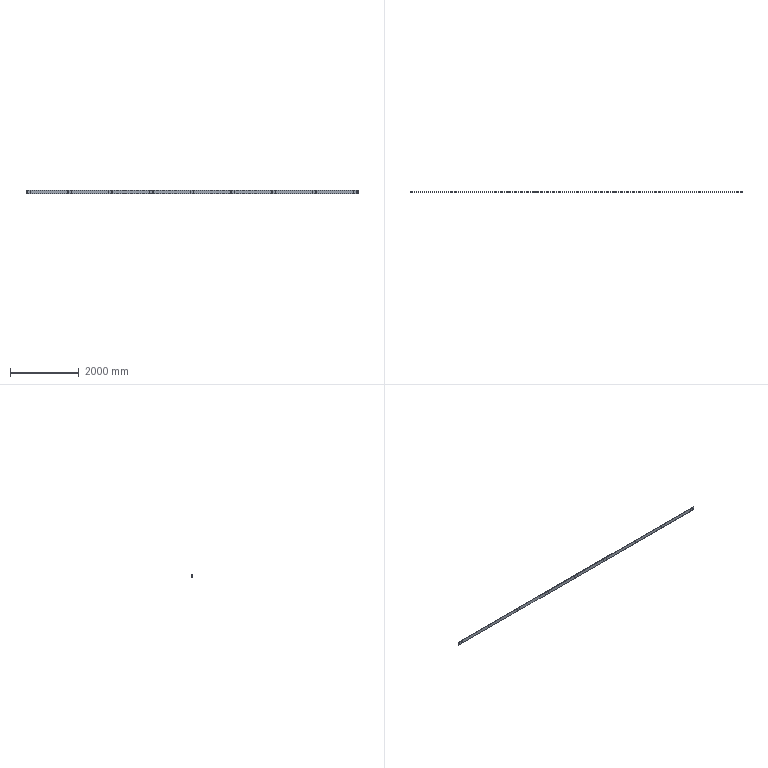Component | SolidWorks | Kick1-1 | 1 solid | 78 faces | volume 9655788 mm3 | cylinder 72 | plane 6 | commonest cylinder face diameters 11 x72 | material Plain Carbon Steel